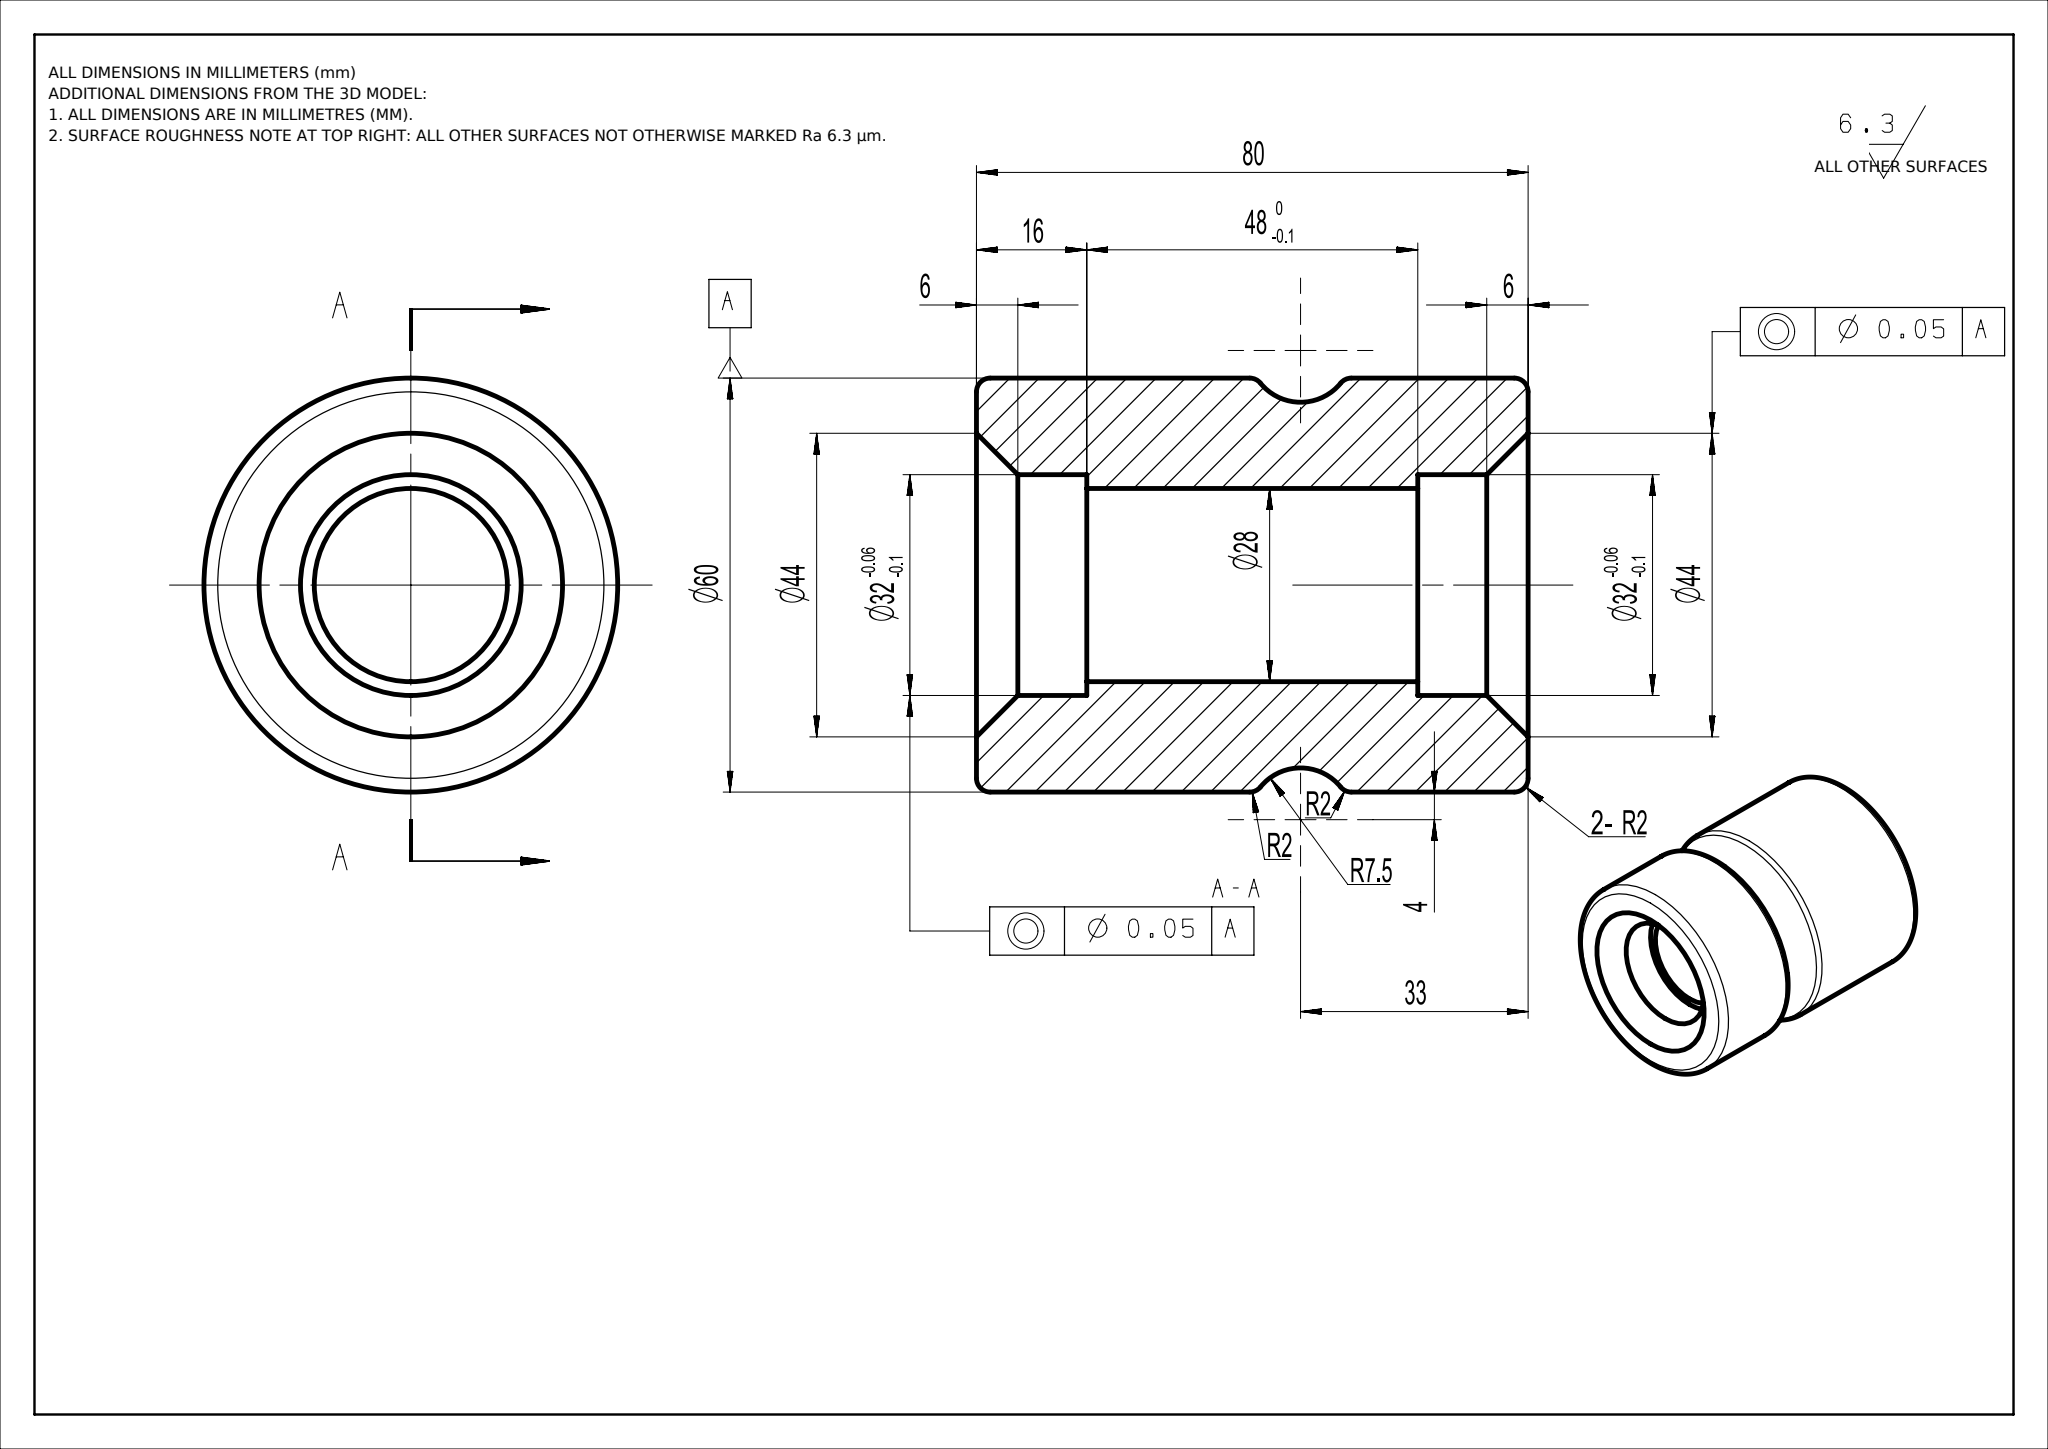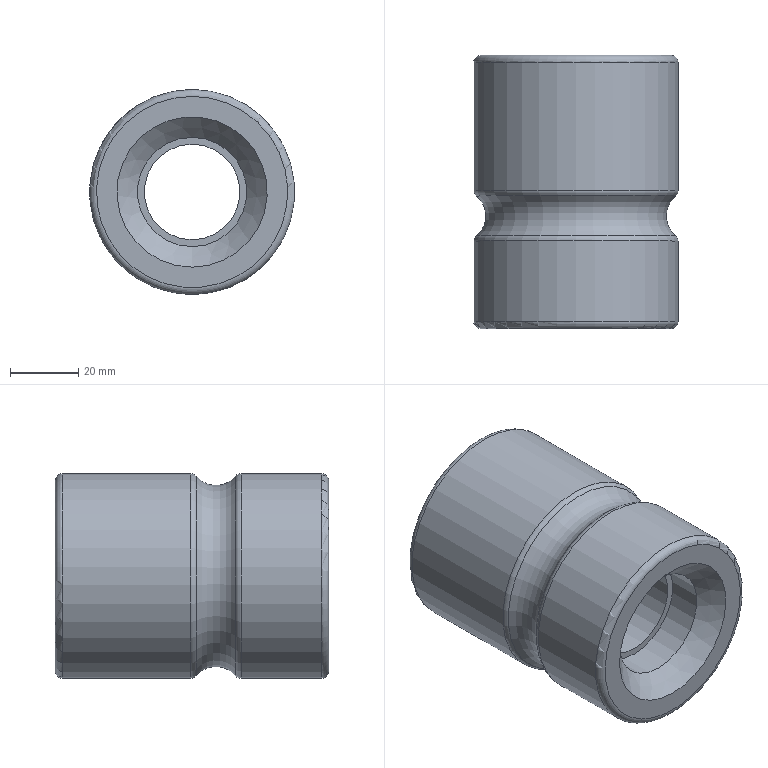Part | NX | mm | 1 solid | 16 faces | box 60 x 80 x 60 mm | volume 160833 mm3 | cylinder 5 | torus 5 | plane 4 | cone 2 | commonest cylinder face diameters 60 x2 32 x2 28 x1
STEP:
#1=CARTESIAN_POINT('',(0.,0.,0.));
#2=DIRECTION('',(0.,0.,1.));
#3=DIRECTION('',(1.,0.,0.));
#4=AXIS2_PLACEMENT_3D('',#1,#2,#3);
#5=(LENGTH_UNIT()NAMED_UNIT(*)SI_UNIT(.MILLI.,.METRE.));
#6=UNCERTAINTY_MEASURE_WITH_UNIT(LENGTH_MEASURE(0.00002),#5,'','');
#7=(NAMED_UNIT(*)PLANE_ANGLE_UNIT()SI_UNIT($,.RADIAN.));
#8=PLANE_ANGLE_MEASURE_WITH_UNIT(PLANE_ANGLE_MEASURE(0.01745),#7);
#9=DIMENSIONAL_EXPONENTS(0.,0.,0.,0.,0.,0.,0.);
#10=(CONVERSION_BASED_UNIT('',#8)NAMED_UNIT(#9)PLANE_ANGLE_UNIT());
#11=(NAMED_UNIT(*)SI_UNIT($,.STERADIAN.)SOLID_ANGLE_UNIT());
#12=(GEOMETRIC_REPRESENTATION_CONTEXT(3)GLOBAL_UNCERTAINTY_ASSIGNED_CONTEXT((#6))GLOBAL_UNIT_ASSIGNED_CONTEXT((#5,#10,#11))REPRESENTATION_CONTEXT('',''));
#13=SHAPE_REPRESENTATION('',(#4),#12);
#14=CARTESIAN_POINT('',(0.,25.635,-30.));
#15=VERTEX_POINT('',#14);
#16=CARTESIAN_POINT('',(0.,25.635,0.));
#17=DIRECTION('',(0.,-1.,0.));
#18=DIRECTION('',(0.,0.,-1.));
#19=AXIS2_PLACEMENT_3D('',#16,#17,#18);
#20=CIRCLE('',#19,30.);
#21=EDGE_CURVE('',#15,#15,#20,.T.);
#22=ORIENTED_EDGE('',*,*,#21,.T.);
#23=EDGE_LOOP('',(#22));
#24=FACE_BOUND('',#23,.T.);
#25=CARTESIAN_POINT('',(0.,2.,30.));
#26=VERTEX_POINT('',#25);
#27=CARTESIAN_POINT('',(0.,2.,0.));
#28=DIRECTION('',(0.,1.,0.));
#29=DIRECTION('',(0.,0.,1.));
#30=AXIS2_PLACEMENT_3D('',#27,#28,#29);
#31=CIRCLE('',#30,30.);
#32=EDGE_CURVE('',#26,#26,#31,.T.);
#33=ORIENTED_EDGE('',*,*,#32,.T.);
#34=EDGE_LOOP('',(#33));
#35=FACE_BOUND('',#34,.T.);
#36=CARTESIAN_POINT('',(0.,0.,0.));
#37=DIRECTION('',(0.,-1.,0.));
#38=DIRECTION('',(0.,0.,-1.));
#39=AXIS2_PLACEMENT_3D('',#36,#37,#38);
#40=CYLINDRICAL_SURFACE('',#39,30.);
#41=ADVANCED_FACE('',(#24,#35),#40,.T.);
#42=CARTESIAN_POINT('',(0.,40.365,30.));
#43=VERTEX_POINT('',#42);
#44=CARTESIAN_POINT('',(0.,40.365,0.));
#45=DIRECTION('',(0.,1.,0.));
#46=DIRECTION('',(0.,0.,1.));
#47=AXIS2_PLACEMENT_3D('',#44,#45,#46);
#48=CIRCLE('',#47,30.);
#49=EDGE_CURVE('',#43,#43,#48,.T.);
#50=ORIENTED_EDGE('',*,*,#49,.T.);
#51=EDGE_LOOP('',(#50));
#52=FACE_BOUND('',#51,.T.);
#53=CARTESIAN_POINT('',(0.,78.,-30.));
#54=VERTEX_POINT('',#53);
#55=CARTESIAN_POINT('',(0.,78.,0.));
#56=DIRECTION('',(0.,-1.,0.));
#57=DIRECTION('',(0.,0.,-1.));
#58=AXIS2_PLACEMENT_3D('',#55,#56,#57);
#59=CIRCLE('',#58,30.);
#60=EDGE_CURVE('',#54,#54,#59,.T.);
#61=ORIENTED_EDGE('',*,*,#60,.T.);
#62=EDGE_LOOP('',(#61));
#63=FACE_BOUND('',#62,.T.);
#64=CARTESIAN_POINT('',(0.,0.,0.));
#65=DIRECTION('',(0.,-1.,0.));
#66=DIRECTION('',(0.,0.,-1.));
#67=AXIS2_PLACEMENT_3D('',#64,#65,#66);
#68=CYLINDRICAL_SURFACE('',#67,30.);
#69=ADVANCED_FACE('',(#52,#63),#68,.T.);
#70=CARTESIAN_POINT('',(0.,0.,28.));
#71=VERTEX_POINT('',#70);
#72=CARTESIAN_POINT('',(0.,0.,0.));
#73=DIRECTION('',(0.,-1.,0.));
#74=DIRECTION('',(0.,0.,1.));
#75=AXIS2_PLACEMENT_3D('',#72,#73,#74);
#76=CIRCLE('',#75,28.);
#77=EDGE_CURVE('',#71,#71,#76,.T.);
#78=ORIENTED_EDGE('',*,*,#77,.T.);
#79=EDGE_LOOP('',(#78));
#80=FACE_BOUND('',#79,.T.);
#81=CARTESIAN_POINT('',(0.,0.,-22.));
#82=VERTEX_POINT('',#81);
#83=CARTESIAN_POINT('',(0.,0.,0.));
#84=DIRECTION('',(0.,-1.,0.));
#85=DIRECTION('',(0.,0.,-1.));
#86=AXIS2_PLACEMENT_3D('',#83,#84,#85);
#87=CIRCLE('',#86,22.);
#88=EDGE_CURVE('',#82,#82,#87,.T.);
#89=ORIENTED_EDGE('',*,*,#88,.F.);
#90=EDGE_LOOP('',(#89));
#91=FACE_BOUND('',#90,.T.);
#92=CARTESIAN_POINT('',(0.,0.,30.));
#93=DIRECTION('',(0.,1.,0.));
#94=DIRECTION('',(0.,0.,1.));
#95=AXIS2_PLACEMENT_3D('',#92,#93,#94);
#96=PLANE('',#95);
#97=ADVANCED_FACE('',(#80,#91),#96,.F.);
#98=CARTESIAN_POINT('',(0.,6.,-16.));
#99=VERTEX_POINT('',#98);
#100=CARTESIAN_POINT('',(0.,6.,0.));
#101=DIRECTION('',(0.,-1.,0.));
#102=DIRECTION('',(0.,0.,-1.));
#103=AXIS2_PLACEMENT_3D('',#100,#101,#102);
#104=CIRCLE('',#103,16.);
#105=EDGE_CURVE('',#99,#99,#104,.T.);
#106=ORIENTED_EDGE('',*,*,#105,.F.);
#107=EDGE_LOOP('',(#106));
#108=FACE_BOUND('',#107,.T.);
#109=ORIENTED_EDGE('',*,*,#88,.T.);
#110=EDGE_LOOP('',(#109));
#111=FACE_BOUND('',#110,.T.);
#112=CARTESIAN_POINT('',(0.,0.,0.));
#113=DIRECTION('',(0.,-1.,0.));
#114=DIRECTION('',(0.,0.,-1.));
#115=AXIS2_PLACEMENT_3D('',#112,#113,#114);
#116=CONICAL_SURFACE('',#115,22.,45.);
#117=ADVANCED_FACE('',(#108,#111),#116,.F.);
#118=CARTESIAN_POINT('',(0.,16.,-16.));
#119=VERTEX_POINT('',#118);
#120=CARTESIAN_POINT('',(0.,16.,0.));
#121=DIRECTION('',(0.,-1.,0.));
#122=DIRECTION('',(0.,0.,-1.));
#123=AXIS2_PLACEMENT_3D('',#120,#121,#122);
#124=CIRCLE('',#123,16.);
#125=EDGE_CURVE('',#119,#119,#124,.T.);
#126=ORIENTED_EDGE('',*,*,#125,.F.);
#127=EDGE_LOOP('',(#126));
#128=FACE_BOUND('',#127,.T.);
#129=ORIENTED_EDGE('',*,*,#105,.T.);
#130=EDGE_LOOP('',(#129));
#131=FACE_BOUND('',#130,.T.);
#132=CARTESIAN_POINT('',(0.,0.,0.));
#133=DIRECTION('',(0.,-1.,0.));
#134=DIRECTION('',(0.,0.,-1.));
#135=AXIS2_PLACEMENT_3D('',#132,#133,#134);
#136=CYLINDRICAL_SURFACE('',#135,16.);
#137=ADVANCED_FACE('',(#128,#131),#136,.F.);
#138=CARTESIAN_POINT('',(0.,16.,-14.));
#139=VERTEX_POINT('',#138);
#140=CARTESIAN_POINT('',(0.,16.,0.));
#141=DIRECTION('',(0.,-1.,0.));
#142=DIRECTION('',(0.,0.,-1.));
#143=AXIS2_PLACEMENT_3D('',#140,#141,#142);
#144=CIRCLE('',#143,14.);
#145=EDGE_CURVE('',#139,#139,#144,.T.);
#146=ORIENTED_EDGE('',*,*,#145,.F.);
#147=EDGE_LOOP('',(#146));
#148=FACE_BOUND('',#147,.T.);
#149=ORIENTED_EDGE('',*,*,#125,.T.);
#150=EDGE_LOOP('',(#149));
#151=FACE_BOUND('',#150,.T.);
#152=CARTESIAN_POINT('',(0.,16.,16.));
#153=DIRECTION('',(0.,1.,0.));
#154=DIRECTION('',(0.,0.,1.));
#155=AXIS2_PLACEMENT_3D('',#152,#153,#154);
#156=PLANE('',#155);
#157=ADVANCED_FACE('',(#148,#151),#156,.F.);
#158=CARTESIAN_POINT('',(0.,64.,-14.));
#159=VERTEX_POINT('',#158);
#160=CARTESIAN_POINT('',(0.,64.,0.));
#161=DIRECTION('',(0.,-1.,0.));
#162=DIRECTION('',(0.,0.,-1.));
#163=AXIS2_PLACEMENT_3D('',#160,#161,#162);
#164=CIRCLE('',#163,14.);
#165=EDGE_CURVE('',#159,#159,#164,.T.);
#166=ORIENTED_EDGE('',*,*,#165,.F.);
#167=EDGE_LOOP('',(#166));
#168=FACE_BOUND('',#167,.T.);
#169=ORIENTED_EDGE('',*,*,#145,.T.);
#170=EDGE_LOOP('',(#169));
#171=FACE_BOUND('',#170,.T.);
#172=CARTESIAN_POINT('',(0.,0.,0.));
#173=DIRECTION('',(0.,-1.,0.));
#174=DIRECTION('',(0.,0.,-1.));
#175=AXIS2_PLACEMENT_3D('',#172,#173,#174);
#176=CYLINDRICAL_SURFACE('',#175,14.);
#177=ADVANCED_FACE('',(#168,#171),#176,.F.);
#178=CARTESIAN_POINT('',(0.,64.,-16.));
#179=VERTEX_POINT('',#178);
#180=CARTESIAN_POINT('',(0.,64.,0.));
#181=DIRECTION('',(0.,-1.,0.));
#182=DIRECTION('',(0.,0.,-1.));
#183=AXIS2_PLACEMENT_3D('',#180,#181,#182);
#184=CIRCLE('',#183,16.);
#185=EDGE_CURVE('',#179,#179,#184,.T.);
#186=ORIENTED_EDGE('',*,*,#185,.F.);
#187=EDGE_LOOP('',(#186));
#188=FACE_BOUND('',#187,.T.);
#189=ORIENTED_EDGE('',*,*,#165,.T.);
#190=EDGE_LOOP('',(#189));
#191=FACE_BOUND('',#190,.T.);
#192=CARTESIAN_POINT('',(0.,64.,14.));
#193=DIRECTION('',(0.,-1.,0.));
#194=DIRECTION('',(0.,0.,-1.));
#195=AXIS2_PLACEMENT_3D('',#192,#193,#194);
#196=PLANE('',#195);
#197=ADVANCED_FACE('',(#188,#191),#196,.F.);
#198=CARTESIAN_POINT('',(0.,74.,-16.));
#199=VERTEX_POINT('',#198);
#200=CARTESIAN_POINT('',(0.,74.,0.));
#201=DIRECTION('',(0.,-1.,0.));
#202=DIRECTION('',(0.,0.,-1.));
#203=AXIS2_PLACEMENT_3D('',#200,#201,#202);
#204=CIRCLE('',#203,16.);
#205=EDGE_CURVE('',#199,#199,#204,.T.);
#206=ORIENTED_EDGE('',*,*,#205,.F.);
#207=EDGE_LOOP('',(#206));
#208=FACE_BOUND('',#207,.T.);
#209=ORIENTED_EDGE('',*,*,#185,.T.);
#210=EDGE_LOOP('',(#209));
#211=FACE_BOUND('',#210,.T.);
#212=CARTESIAN_POINT('',(0.,0.,0.));
#213=DIRECTION('',(0.,-1.,0.));
#214=DIRECTION('',(0.,0.,-1.));
#215=AXIS2_PLACEMENT_3D('',#212,#213,#214);
#216=CYLINDRICAL_SURFACE('',#215,16.);
#217=ADVANCED_FACE('',(#208,#211),#216,.F.);
#218=CARTESIAN_POINT('',(0.,80.,-22.));
#219=VERTEX_POINT('',#218);
#220=CARTESIAN_POINT('',(0.,80.,0.));
#221=DIRECTION('',(0.,-1.,0.));
#222=DIRECTION('',(0.,0.,-1.));
#223=AXIS2_PLACEMENT_3D('',#220,#221,#222);
#224=CIRCLE('',#223,22.);
#225=EDGE_CURVE('',#219,#219,#224,.T.);
#226=ORIENTED_EDGE('',*,*,#225,.F.);
#227=EDGE_LOOP('',(#226));
#228=FACE_BOUND('',#227,.T.);
#229=ORIENTED_EDGE('',*,*,#205,.T.);
#230=EDGE_LOOP('',(#229));
#231=FACE_BOUND('',#230,.T.);
#232=CARTESIAN_POINT('',(0.,74.,0.));
#233=DIRECTION('',(0.,1.,0.));
#234=DIRECTION('',(0.,0.,1.));
#235=AXIS2_PLACEMENT_3D('',#232,#233,#234);
#236=CONICAL_SURFACE('',#235,16.,45.);
#237=ADVANCED_FACE('',(#228,#231),#236,.F.);
#238=CARTESIAN_POINT('',(0.,80.,-28.));
#239=VERTEX_POINT('',#238);
#240=CARTESIAN_POINT('',(0.,80.,0.));
#241=DIRECTION('',(0.,1.,0.));
#242=DIRECTION('',(0.,0.,-1.));
#243=AXIS2_PLACEMENT_3D('',#240,#241,#242);
#244=CIRCLE('',#243,28.);
#245=EDGE_CURVE('',#239,#239,#244,.T.);
#246=ORIENTED_EDGE('',*,*,#245,.T.);
#247=EDGE_LOOP('',(#246));
#248=FACE_BOUND('',#247,.T.);
#249=ORIENTED_EDGE('',*,*,#225,.T.);
#250=EDGE_LOOP('',(#249));
#251=FACE_BOUND('',#250,.T.);
#252=CARTESIAN_POINT('',(0.,80.,22.));
#253=DIRECTION('',(0.,-1.,0.));
#254=DIRECTION('',(0.,0.,-1.));
#255=AXIS2_PLACEMENT_3D('',#252,#253,#254);
#256=PLANE('',#255);
#257=ADVANCED_FACE('',(#248,#251),#256,.F.);
#258=ORIENTED_EDGE('',*,*,#245,.F.);
#259=EDGE_LOOP('',(#258));
#260=FACE_BOUND('',#259,.T.);
#261=ORIENTED_EDGE('',*,*,#60,.F.);
#262=EDGE_LOOP('',(#261));
#263=FACE_BOUND('',#262,.T.);
#264=CARTESIAN_POINT('',(0.,78.,0.));
#265=DIRECTION('',(0.,-1.,0.));
#266=DIRECTION('',(0.,0.,-1.));
#267=AXIS2_PLACEMENT_3D('',#264,#265,#266);
#268=TOROIDAL_SURFACE('',#267,28.,2.);
#269=ADVANCED_FACE('',(#260,#263),#268,.T.);
#270=ORIENTED_EDGE('',*,*,#32,.F.);
#271=EDGE_LOOP('',(#270));
#272=FACE_BOUND('',#271,.T.);
#273=ORIENTED_EDGE('',*,*,#77,.F.);
#274=EDGE_LOOP('',(#273));
#275=FACE_BOUND('',#274,.T.);
#276=CARTESIAN_POINT('',(0.,2.,0.));
#277=DIRECTION('',(0.,1.,0.));
#278=DIRECTION('',(0.,0.,1.));
#279=AXIS2_PLACEMENT_3D('',#276,#277,#278);
#280=TOROIDAL_SURFACE('',#279,28.,2.);
#281=ADVANCED_FACE('',(#272,#275),#280,.T.);
#282=CARTESIAN_POINT('',(0.,38.815,-29.263));
#283=VERTEX_POINT('',#282);
#284=CARTESIAN_POINT('',(0.,38.815,0.));
#285=DIRECTION('',(0.,-1.,0.));
#286=DIRECTION('',(0.,0.,-1.));
#287=AXIS2_PLACEMENT_3D('',#284,#285,#286);
#288=CIRCLE('',#287,29.263);
#289=EDGE_CURVE('',#283,#283,#288,.T.);
#290=ORIENTED_EDGE('',*,*,#289,.T.);
#291=EDGE_LOOP('',(#290));
#292=FACE_BOUND('',#291,.T.);
#293=CARTESIAN_POINT('',(0.,27.185,29.263));
#294=VERTEX_POINT('',#293);
#295=CARTESIAN_POINT('',(0.,27.185,0.));
#296=DIRECTION('',(0.,1.,0.));
#297=DIRECTION('',(0.,0.,1.));
#298=AXIS2_PLACEMENT_3D('',#295,#296,#297);
#299=CIRCLE('',#298,29.263);
#300=EDGE_CURVE('',#294,#294,#299,.T.);
#301=ORIENTED_EDGE('',*,*,#300,.T.);
#302=EDGE_LOOP('',(#301));
#303=FACE_BOUND('',#302,.T.);
#304=CARTESIAN_POINT('',(0.,33.,0.));
#305=DIRECTION('',(0.,-1.,0.));
#306=DIRECTION('',(0.,0.,-1.));
#307=AXIS2_PLACEMENT_3D('',#304,#305,#306);
#308=TOROIDAL_SURFACE('',#307,34.,7.5);
#309=ADVANCED_FACE('',(#292,#303),#308,.F.);
#310=ORIENTED_EDGE('',*,*,#49,.F.);
#311=EDGE_LOOP('',(#310));
#312=FACE_BOUND('',#311,.T.);
#313=ORIENTED_EDGE('',*,*,#289,.F.);
#314=EDGE_LOOP('',(#313));
#315=FACE_BOUND('',#314,.T.);
#316=CARTESIAN_POINT('',(0.,40.365,0.));
#317=DIRECTION('',(0.,1.,0.));
#318=DIRECTION('',(0.,0.,1.));
#319=AXIS2_PLACEMENT_3D('',#316,#317,#318);
#320=TOROIDAL_SURFACE('',#319,28.,2.);
#321=ADVANCED_FACE('',(#312,#315),#320,.T.);
#322=ORIENTED_EDGE('',*,*,#21,.F.);
#323=EDGE_LOOP('',(#322));
#324=FACE_BOUND('',#323,.T.);
#325=ORIENTED_EDGE('',*,*,#300,.F.);
#326=EDGE_LOOP('',(#325));
#327=FACE_BOUND('',#326,.T.);
#328=CARTESIAN_POINT('',(0.,25.635,0.));
#329=DIRECTION('',(0.,-1.,0.));
#330=DIRECTION('',(0.,0.,-1.));
#331=AXIS2_PLACEMENT_3D('',#328,#329,#330);
#332=TOROIDAL_SURFACE('',#331,28.,2.);
#333=ADVANCED_FACE('',(#324,#327),#332,.T.);
#334=CLOSED_SHELL('',(#41,#69,#97,#117,#137,#157,#177,#197,#217,#237,#257,#269,#281,#309,#321,#333));
#335=MANIFOLD_SOLID_BREP('',#334);
#336=ADVANCED_BREP_SHAPE_REPRESENTATION('',(#335),#12);
#337=SHAPE_REPRESENTATION_RELATIONSHIP('','',#13,#336);
#338=PRESENTATION_LAYER_ASSIGNMENT('','',(#335));
#339=COLOUR_RGB('',0.2,0.2,1.);
#340=FILL_AREA_STYLE_COLOUR('',#339);
#341=FILL_AREA_STYLE('',(#340));
#342=SURFACE_STYLE_FILL_AREA(#341);
#343=SURFACE_SIDE_STYLE('',(#342));
#344=SURFACE_STYLE_USAGE(.BOTH.,#343);
#345=PRESENTATION_STYLE_ASSIGNMENT((#344));
#346=STYLED_ITEM('',(#345),#335);
#347=MECHANICAL_DESIGN_GEOMETRIC_PRESENTATION_REPRESENTATION('',(#346),#12);